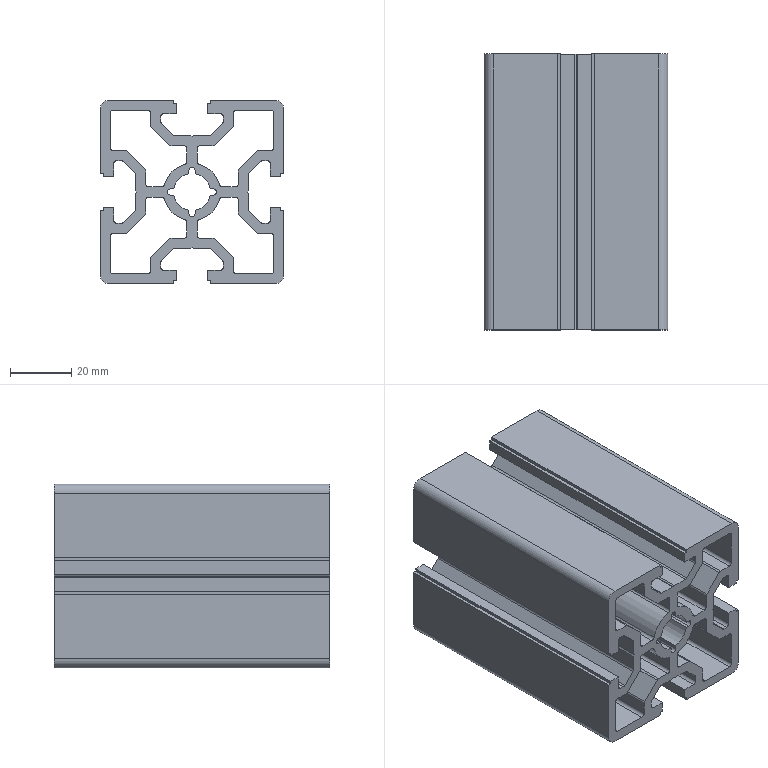Component | SolidWorks | AOB02-H6060YE-L90-1 | 1 solid | 207 faces | volume 123309 mm3 | plane 122 | cylinder 85 | commonest cylinder face diameters 2 x73 6 x4 18.6 x4 12 x4